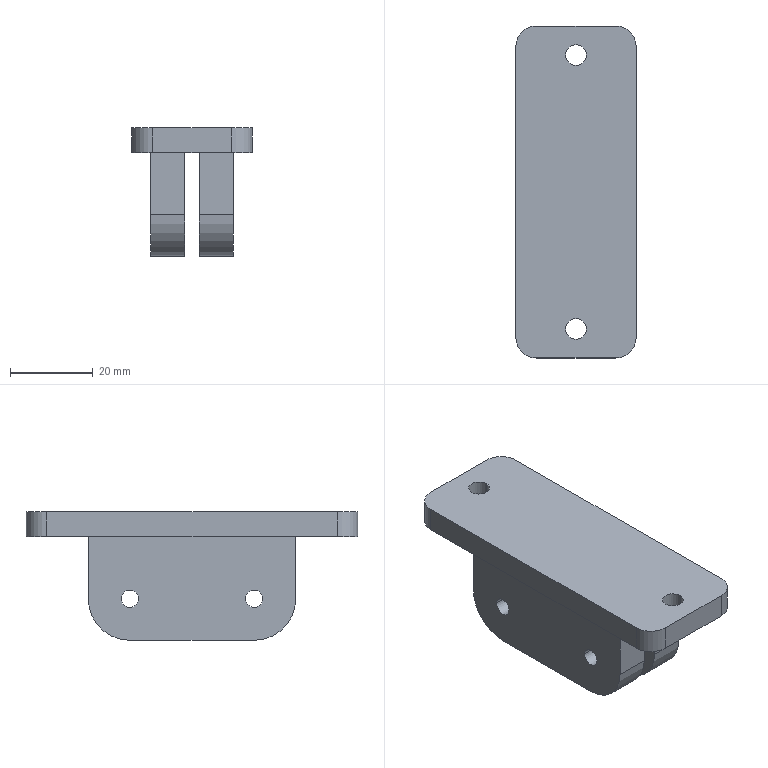Component | SolidWorks | CutterFixingBlock-1 | 1 solid | 36 faces | box 29 x 80 x 31 mm | volume 32852 mm3 | cylinder 20 | plane 16 | commonest cylinder face diameters 4.2 x4 5.5 x4 5 x4 20 x4 10 x4 | material 1060 Alloy
build123d program:
from build123d import *

# Parameters (mm, degrees)
SKETCH1_W                = 80
SKETCH1_H                = 6
BOSS_EXTRUDE1_DEPTH      = 14.5
F_5_0_5_DIAMETER_HOLE1_D = 5
SKETCH5_W                = 50
SKETCH5_H                = 20
BOSS_EXTRUDE2_DEPTH      = 25
FILLET1_R                = 5
FILLET2_R                = 10
CUT_EXTRUDE1_START       = -25
SKETCH6_W                = 50
SKETCH6_H                = 3.5
CUT_EXTRUDE1_DEPTH       = 25
SKETCH7_R                = 2.75
CUT_EXTRUDE2_DEPTH       = 8.25
M5_TAPPED_HOLE1_D        = 4.2


with BuildPart() as part:
    # Sketch1 → Boss-Extrude1 (new, symmetric)
    with BuildSketch(Plane.XY):
        with Locations((0, -3)):
            Rectangle(SKETCH1_W, SKETCH1_H)
    extrude(amount=BOSS_EXTRUDE1_DEPTH, both=True)

    # 5.0 _5_ Diameter Hole1 (through all)
    with Locations(Plane(origin=(0, 0, 0), x_dir=(1, 0, 0), z_dir=(0, 1, 0))):
        with Locations((-33, 0), (33, 0)):
            Hole(F_5_0_5_DIAMETER_HOLE1_D / 2)

    # Sketch5 → Boss-Extrude2 (add)
    with BuildSketch(Plane(origin=(0, 0, 0), x_dir=(1, 0, 0), z_dir=(0, 1, 0))):
        Rectangle(SKETCH5_W, SKETCH5_H)
    extrude(amount=BOSS_EXTRUDE2_DEPTH)

    # Fillet1
    fillet1_edges = [part.edges().sort_by_distance(p)[0] for p in [
        (40, -3, 14.5),
        (-40, -3, 14.5),
        (40, -3, -14.5),
        (-40, -3, -14.5),
    ]]
    fillet(fillet1_edges, radius=FILLET1_R)

    # Fillet2
    fillet2_edges = [part.edges().sort_by_distance(p)[0] for p in [
        (-25, 25, 0),
        (25, 25, 0),
    ]]
    fillet(fillet2_edges, radius=FILLET2_R)

    # Sketch6 → Cut-Extrude1 (cut)
    with BuildSketch(Plane(origin=(0, 25, 0), x_dir=(1, 0, 0), z_dir=(0, 1, 0)).offset(CUT_EXTRUDE1_START)):
        Rectangle(SKETCH6_W, SKETCH6_H)
    extrude(amount=CUT_EXTRUDE1_DEPTH, mode=Mode.SUBTRACT)

    # Sketch7 → Cut-Extrude2 (cut)
    with BuildSketch(Plane.XY.offset(10)):
        with Locations((-15, 15)):
            Circle(SKETCH7_R)
        with Locations((15, 15)):
            Circle(SKETCH7_R)
    extrude(amount=-CUT_EXTRUDE2_DEPTH, mode=Mode.SUBTRACT)

    # M5 Tapped Hole1 (through all)
    with Locations(Plane.XY.offset(-1.75)):
        with Locations((15, 15), (-15, 15)):
            Hole(M5_TAPPED_HOLE1_D / 2)


solid = part.part

# Placed as in the assembly
solid = solid.moved(Location((-194.766, 347.264, 146), (-90, 90, 0)))